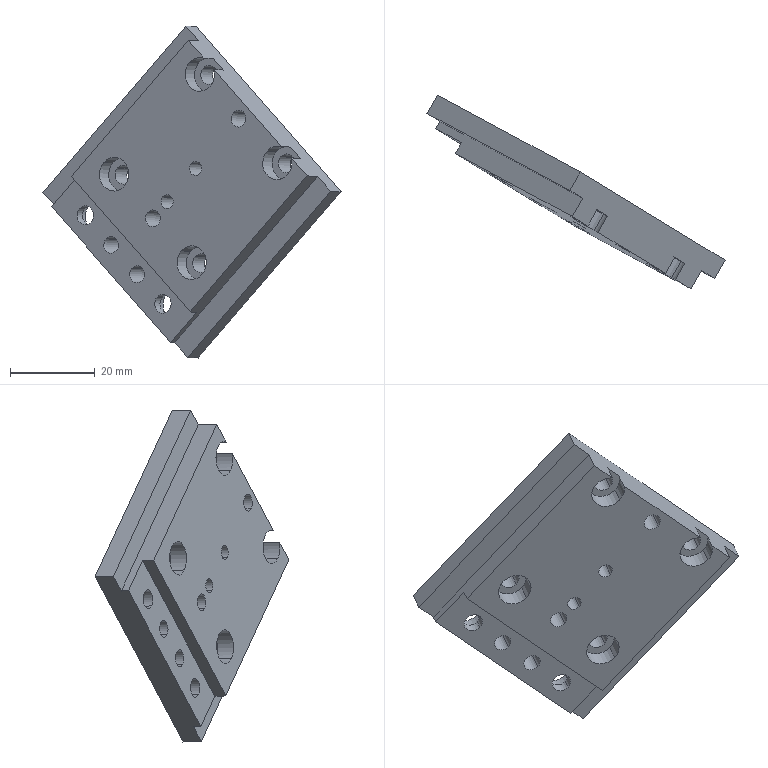Component | SolidWorks | 8z0-123-1 | 1 solid | 56 faces | box 70.56 x 45.89 x 78.58 mm | volume 24310 mm3 | cylinder 38 | plane 18 | commonest cylinder face diameters 8 x14 4.5 x12 4 x8 3.3 x4
build123d program:
from build123d import *

# Parameters (mm, degrees)
SKETCH1_W                                       = 46
SKETCH1_H                                       = 60
BOSS_EXTRUDE1_DEPTH                             = 10
SKETCH2_W                                       = 46
SKETCH2_H                                       = 10
CUT_EXTRUDE1_DEPTH                              = 3
SIZE_MM_DOWEL_PIN_HOLE1_D                       = 4
SIZE_MM_DOWEL_PIN_HOLE1_DEPTH                   = 10
SIZE_MM_DOWEL_PIN_HOLE1_TIP                     = 1.202
M4_HEX_SOCKET_HEAD_CAP_SCREW_CBORE1_D           = 4.5
M4_HEX_SOCKET_HEAD_CAP_SCREW_CBORE1_CBORE_D     = 8
M4_HEX_SOCKET_HEAD_CAP_SCREW_CBORE1_CBORE_DEPTH = 4.5
M4_TAPPED_HOLE1_D                               = 3.3
M4_TAPPED_HOLE1_DEPTH                           = 10.1
M4_TAPPED_HOLE1_TIP                             = 0.9914
SKETCH10_W                                      = 5
SKETCH10_H                                      = 60
BOSS_EXTRUDE3_DEPTH                             = 5
SKETCH12_W                                      = 10
SKETCH12_H                                      = 5
CUT_EXTRUDE3_DEPTH                              = 65.312
SIZE_MM_DOWEL_PIN_HOLE2_D                       = 4
SIZE_MM_DOWEL_PIN_HOLE2_DEPTH                   = 10
SIZE_MM_DOWEL_PIN_HOLE2_TIP                     = 1.202
M4_HEX_SOCKET_HEAD_CAP_SCREW_CBORE2_D           = 4.5
M4_HEX_SOCKET_HEAD_CAP_SCREW_CBORE2_CBORE_D     = 8
M4_HEX_SOCKET_HEAD_CAP_SCREW_CBORE2_CBORE_DEPTH = 4.4


with BuildPart() as part:
    # Sketch1 → Boss-Extrude1 (new body)
    with BuildSketch(Plane.XY):
        Rectangle(SKETCH1_W, SKETCH1_H)
    extrude(amount=BOSS_EXTRUDE1_DEPTH)

    # Sketch2 → Cut-Extrude1 (cut)
    with BuildSketch(Plane.XY.offset(10)):
        with Locations((0, 20)):
            Rectangle(SKETCH2_W, SKETCH2_H)
    extrude(amount=-CUT_EXTRUDE1_DEPTH, mode=Mode.SUBTRACT)

    # Size mm Dowel Pin Hole1
    with Locations(Plane.XY.offset(7)):
        with Locations((-5, 20), (5, 20)):
            Hole(SIZE_MM_DOWEL_PIN_HOLE1_D / 2, depth=SIZE_MM_DOWEL_PIN_HOLE1_DEPTH)
            with Locations((0, 0, -(SIZE_MM_DOWEL_PIN_HOLE1_DEPTH + SIZE_MM_DOWEL_PIN_HOLE1_TIP / 2))):  # 118° drill point
                Cone(0, SIZE_MM_DOWEL_PIN_HOLE1_D / 2, SIZE_MM_DOWEL_PIN_HOLE1_TIP, mode=Mode.SUBTRACT)

    # M4 Hex Socket Head Cap Screw CBORE1 (through all)
    with Locations(Plane(origin=(0, 0, 0), x_dir=(-1, 0, 0), z_dir=(0, 0, -1))):
        with Locations((-15, 20), (15, 20)):
            CounterBoreHole(M4_HEX_SOCKET_HEAD_CAP_SCREW_CBORE1_D / 2, M4_HEX_SOCKET_HEAD_CAP_SCREW_CBORE1_CBORE_D / 2, M4_HEX_SOCKET_HEAD_CAP_SCREW_CBORE1_CBORE_DEPTH)

    # M4 Tapped Hole1
    with Locations(Plane.XY.offset(10)):
        with Locations((0, -10), (0, 1)):
            Hole(M4_TAPPED_HOLE1_D / 2, depth=M4_TAPPED_HOLE1_DEPTH)
            with Locations((0, 0, -(M4_TAPPED_HOLE1_DEPTH + M4_TAPPED_HOLE1_TIP / 2))):  # 118° drill point
                Cone(0, M4_TAPPED_HOLE1_D / 2, M4_TAPPED_HOLE1_TIP, mode=Mode.SUBTRACT)

    # Sketch10 → Boss-Extrude3 (add)
    with BuildSketch(Plane.ZY.offset(23)):
        with Locations((2.5, 0)):
            Rectangle(SKETCH10_W, SKETCH10_H)
    boss_extrude3 = extrude(amount=BOSS_EXTRUDE3_DEPTH)

    # Mirror2: Boss-Extrude3 across plane
    add(boss_extrude3.mirror(Plane(origin=(0, 0, 0), x_dir=(0, 0, 1), z_dir=(1, 0, 0))))

    # Sketch12 → Cut-Extrude3 (cut, through all)
    with BuildSketch(Plane(origin=(28, 0, 0), x_dir=(0, 0, -1), z_dir=(1, 0, 0))):
        with Locations((-5, 27.5)):
            Rectangle(SKETCH12_W, SKETCH12_H)
    extrude(amount=-CUT_EXTRUDE3_DEPTH, mode=Mode.SUBTRACT)

    # Size mm Dowel Pin Hole2
    with Locations(Plane.XY.offset(10)):
        with Locations((0, -26.5), (0, 6.5)):
            Hole(SIZE_MM_DOWEL_PIN_HOLE2_D / 2, depth=SIZE_MM_DOWEL_PIN_HOLE2_DEPTH)
            with Locations((0, 0, -(SIZE_MM_DOWEL_PIN_HOLE2_DEPTH + SIZE_MM_DOWEL_PIN_HOLE2_TIP / 2))):  # 118° drill point
                Cone(0, SIZE_MM_DOWEL_PIN_HOLE2_D / 2, SIZE_MM_DOWEL_PIN_HOLE2_TIP, mode=Mode.SUBTRACT)

    # M4 Hex Socket Head Cap Screw CBORE2 (through all)
    with Locations(Plane.XY.offset(10)):
        with Locations((-15, 6.5), (15, 6.5), (15, -26.5), (-15, -26.5)):
            CounterBoreHole(M4_HEX_SOCKET_HEAD_CAP_SCREW_CBORE2_D / 2, M4_HEX_SOCKET_HEAD_CAP_SCREW_CBORE2_CBORE_D / 2, M4_HEX_SOCKET_HEAD_CAP_SCREW_CBORE2_CBORE_DEPTH)


solid = part.part

# Placed as in the assembly
solid = solid.moved(Location((47.285, -37.769, 163.843), (88.336, -29.849, 134.87)))